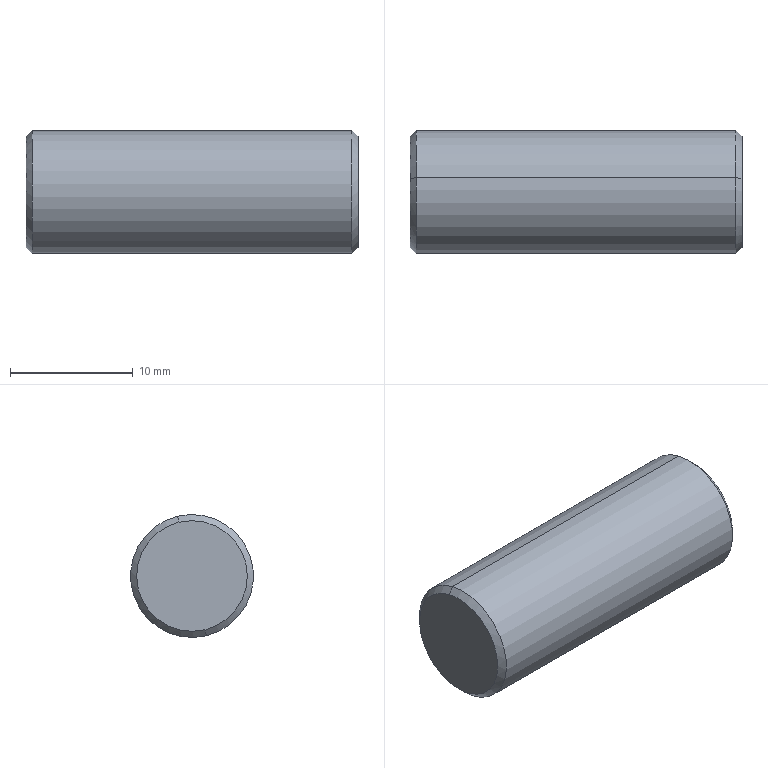Component | SolidWorks | STB-08-015-1 | 1 solid | 8 faces | box 27 x 10 x 10 mm | volume 2113 mm3 | cone 4 | cylinder 2 | plane 2 | commonest cylinder face diameters 10 x2
build123d program:
from build123d import *

# Parameters (mm, degrees)
SKETCH1_R           = 5
BOSS_EXTRUDE1_DEPTH = 13.5
CHAMFER1_SIZE       = 0.5


with BuildPart() as part:
    # Sketch1 → Boss-Extrude1 (new, symmetric)
    with BuildSketch(Plane(origin=(0, 0, 0), x_dir=(0, 0, -1), z_dir=(1, 0, 0))):
        Circle(SKETCH1_R)
    extrude(amount=BOSS_EXTRUDE1_DEPTH, both=True)

    # Chamfer1
    chamfer1_edges = [part.edges().sort_by_distance(p)[0] for p in [
        (-13.5, 0, 5),
        (13.5, 0, 5),
    ]]
    chamfer(chamfer1_edges, length=CHAMFER1_SIZE)


solid = part.part

# Placed as in the assembly
solid = solid.moved(Location((-241.404, 211.999, 2), (0, 0, 0)))
STEP:
#1=CARTESIAN_POINT('',(-8.973,8.388,0.251));
#2=VERTEX_POINT('',#1);
#3=CARTESIAN_POINT('',(-8.973,8.305,-0.09347));
#4=VERTEX_POINT('',#3);
#5=CARTESIAN_POINT('',(-8.973,8.346,0.07874));
#6=DIRECTION('',(1.,0.,0.));
#7=DIRECTION('',(0.,0.2348,0.972));
#8=AXIS2_PLACEMENT_3D('',#5,#6,#7);
#9=CIRCLE('',#8,0.1772);
#10=EDGE_CURVE('',#2,#4,#9,.T.);
#11=ORIENTED_EDGE('',*,*,#10,.F.);
#12=CARTESIAN_POINT('',(-8.992,8.393,0.2701));
#13=VERTEX_POINT('',#12);
#14=CARTESIAN_POINT('',(-8.973,8.388,0.251));
#15=DIRECTION('',(-0.7071,0.166,0.6873));
#16=VECTOR('',#15,39.37);
#17=LINE('',#14,#16);
#18=EDGE_CURVE('',#2,#13,#17,.T.);
#19=ORIENTED_EDGE('',*,*,#18,.T.);
#20=CARTESIAN_POINT('',(-8.992,8.3,-0.1126));
#21=VERTEX_POINT('',#20);
#22=CARTESIAN_POINT('',(-8.992,8.346,0.07874));
#23=DIRECTION('',(-1.,0.,0.));
#24=DIRECTION('',(0.,0.2348,0.972));
#25=AXIS2_PLACEMENT_3D('',#22,#23,#24);
#26=CIRCLE('',#25,0.1969);
#27=EDGE_CURVE('',#21,#13,#26,.T.);
#28=ORIENTED_EDGE('',*,*,#27,.F.);
#29=CARTESIAN_POINT('',(-8.973,8.305,-0.09347));
#30=DIRECTION('',(-0.7071,-0.166,-0.6873));
#31=VECTOR('',#30,39.37);
#32=LINE('',#29,#31);
#33=EDGE_CURVE('',#4,#21,#32,.T.);
#34=ORIENTED_EDGE('',*,*,#33,.F.);
#35=EDGE_LOOP('',(#11,#19,#28,#34));
#36=FACE_OUTER_BOUND('',#35,.T.);
#37=CARTESIAN_POINT('',(-8.973,8.346,0.07874));
#38=DIRECTION('',(-1.,0.,0.));
#39=DIRECTION('',(0.,-0.2348,-0.972));
#40=AXIS2_PLACEMENT_3D('',#37,#38,#39);
#41=CONICAL_SURFACE('',#40,0.1772,0.7854);
#42=ADVANCED_FACE('',(#36),#41,.T.);
#43=CARTESIAN_POINT('',(-10.036,8.305,-0.09347));
#44=VERTEX_POINT('',#43);
#45=CARTESIAN_POINT('',(-10.036,8.388,0.251));
#46=VERTEX_POINT('',#45);
#47=CARTESIAN_POINT('',(-10.036,8.346,0.07874));
#48=DIRECTION('',(-1.,0.,0.));
#49=DIRECTION('',(0.,0.2348,0.972));
#50=AXIS2_PLACEMENT_3D('',#47,#48,#49);
#51=CIRCLE('',#50,0.1772);
#52=EDGE_CURVE('',#44,#46,#51,.T.);
#53=ORIENTED_EDGE('',*,*,#52,.F.);
#54=CARTESIAN_POINT('',(-10.016,8.3,-0.1126));
#55=VERTEX_POINT('',#54);
#56=CARTESIAN_POINT('',(-10.016,8.3,-0.1126));
#57=DIRECTION('',(0.7071,-0.166,-0.6873));
#58=VECTOR('',#57,39.37);
#59=LINE('',#56,#58);
#60=EDGE_CURVE('',#44,#55,#59,.T.);
#61=ORIENTED_EDGE('',*,*,#60,.T.);
#62=CARTESIAN_POINT('',(-10.016,8.393,0.2701));
#63=VERTEX_POINT('',#62);
#64=CARTESIAN_POINT('',(-10.016,8.346,0.07874));
#65=DIRECTION('',(1.,0.,0.));
#66=DIRECTION('',(0.,0.2348,0.972));
#67=AXIS2_PLACEMENT_3D('',#64,#65,#66);
#68=CIRCLE('',#67,0.1969);
#69=EDGE_CURVE('',#63,#55,#68,.T.);
#70=ORIENTED_EDGE('',*,*,#69,.F.);
#71=CARTESIAN_POINT('',(-10.016,8.393,0.2701));
#72=DIRECTION('',(0.7071,0.166,0.6873));
#73=VECTOR('',#72,39.37);
#74=LINE('',#71,#73);
#75=EDGE_CURVE('',#46,#63,#74,.T.);
#76=ORIENTED_EDGE('',*,*,#75,.F.);
#77=EDGE_LOOP('',(#53,#61,#70,#76));
#78=FACE_OUTER_BOUND('',#77,.T.);
#79=CARTESIAN_POINT('',(-10.016,8.346,0.07874));
#80=DIRECTION('',(1.,0.,0.));
#81=DIRECTION('',(0.,0.2348,0.972));
#82=AXIS2_PLACEMENT_3D('',#79,#80,#81);
#83=CONICAL_SURFACE('',#82,0.1969,0.7854);
#84=ADVANCED_FACE('',(#78),#83,.T.);
#85=ORIENTED_EDGE('',*,*,#27,.T.);
#86=CARTESIAN_POINT('',(-8.973,8.393,0.2701));
#87=DIRECTION('',(-1.,0.,0.));
#88=VECTOR('',#87,39.37);
#89=LINE('',#86,#88);
#90=EDGE_CURVE('',#13,#63,#89,.T.);
#91=ORIENTED_EDGE('',*,*,#90,.T.);
#92=ORIENTED_EDGE('',*,*,#69,.T.);
#93=CARTESIAN_POINT('',(-8.973,8.3,-0.1126));
#94=DIRECTION('',(-1.,0.,0.));
#95=VECTOR('',#94,39.37);
#96=LINE('',#93,#95);
#97=EDGE_CURVE('',#21,#55,#96,.T.);
#98=ORIENTED_EDGE('',*,*,#97,.F.);
#99=EDGE_LOOP('',(#85,#91,#92,#98));
#100=FACE_OUTER_BOUND('',#99,.T.);
#101=CARTESIAN_POINT('',(-8.973,8.346,0.07874));
#102=DIRECTION('',(-1.,0.,0.));
#103=DIRECTION('',(0.,-0.2348,-0.972));
#104=AXIS2_PLACEMENT_3D('',#101,#102,#103);
#105=CYLINDRICAL_SURFACE('',#104,0.1969);
#106=ADVANCED_FACE('',(#100),#105,.T.);
#107=ORIENTED_EDGE('',*,*,#90,.F.);
#108=CARTESIAN_POINT('',(-8.992,8.346,0.07874));
#109=DIRECTION('',(-1.,0.,0.));
#110=DIRECTION('',(0.,0.2348,0.972));
#111=AXIS2_PLACEMENT_3D('',#108,#109,#110);
#112=CIRCLE('',#111,0.1969);
#113=EDGE_CURVE('',#13,#21,#112,.T.);
#114=ORIENTED_EDGE('',*,*,#113,.T.);
#115=ORIENTED_EDGE('',*,*,#97,.T.);
#116=CARTESIAN_POINT('',(-10.016,8.346,0.07874));
#117=DIRECTION('',(1.,0.,0.));
#118=DIRECTION('',(0.,0.2348,0.972));
#119=AXIS2_PLACEMENT_3D('',#116,#117,#118);
#120=CIRCLE('',#119,0.1969);
#121=EDGE_CURVE('',#55,#63,#120,.T.);
#122=ORIENTED_EDGE('',*,*,#121,.T.);
#123=EDGE_LOOP('',(#107,#114,#115,#122));
#124=FACE_OUTER_BOUND('',#123,.T.);
#125=CARTESIAN_POINT('',(-8.973,8.346,0.07874));
#126=DIRECTION('',(-1.,0.,0.));
#127=DIRECTION('',(0.,-0.2348,-0.972));
#128=AXIS2_PLACEMENT_3D('',#125,#126,#127);
#129=CYLINDRICAL_SURFACE('',#128,0.1969);
#130=ADVANCED_FACE('',(#124),#129,.T.);
#131=CARTESIAN_POINT('',(-8.973,8.346,0.07874));
#132=DIRECTION('',(1.,0.,0.));
#133=DIRECTION('',(0.,0.2348,0.972));
#134=AXIS2_PLACEMENT_3D('',#131,#132,#133);
#135=CIRCLE('',#134,0.1772);
#136=EDGE_CURVE('',#4,#2,#135,.T.);
#137=ORIENTED_EDGE('',*,*,#136,.T.);
#138=ORIENTED_EDGE('',*,*,#10,.T.);
#139=EDGE_LOOP('',(#137,#138));
#140=FACE_OUTER_BOUND('',#139,.T.);
#141=CARTESIAN_POINT('',(-8.973,8.346,0.07874));
#142=DIRECTION('',(1.,0.,0.));
#143=DIRECTION('',(0.,0.2348,0.972));
#144=AXIS2_PLACEMENT_3D('',#141,#142,#143);
#145=PLANE('',#144);
#146=ADVANCED_FACE('',(#140),#145,.T.);
#147=CARTESIAN_POINT('',(-10.036,8.346,0.07874));
#148=DIRECTION('',(-1.,0.,0.));
#149=DIRECTION('',(0.,0.2348,0.972));
#150=AXIS2_PLACEMENT_3D('',#147,#148,#149);
#151=CIRCLE('',#150,0.1772);
#152=EDGE_CURVE('',#46,#44,#151,.T.);
#153=ORIENTED_EDGE('',*,*,#152,.T.);
#154=ORIENTED_EDGE('',*,*,#52,.T.);
#155=EDGE_LOOP('',(#153,#154));
#156=FACE_OUTER_BOUND('',#155,.T.);
#157=CARTESIAN_POINT('',(-10.036,8.346,0.07874));
#158=DIRECTION('',(1.,0.,0.));
#159=DIRECTION('',(0.,0.2348,0.972));
#160=AXIS2_PLACEMENT_3D('',#157,#158,#159);
#161=PLANE('',#160);
#162=ADVANCED_FACE('',(#156),#161,.F.);
#163=ORIENTED_EDGE('',*,*,#60,.F.);
#164=ORIENTED_EDGE('',*,*,#152,.F.);
#165=ORIENTED_EDGE('',*,*,#75,.T.);
#166=ORIENTED_EDGE('',*,*,#121,.F.);
#167=EDGE_LOOP('',(#163,#164,#165,#166));
#168=FACE_OUTER_BOUND('',#167,.T.);
#169=CARTESIAN_POINT('',(-10.016,8.346,0.07874));
#170=DIRECTION('',(1.,0.,0.));
#171=DIRECTION('',(0.,0.2348,0.972));
#172=AXIS2_PLACEMENT_3D('',#169,#170,#171);
#173=CONICAL_SURFACE('',#172,0.1969,0.7854);
#174=ADVANCED_FACE('',(#168),#173,.T.);
#175=ORIENTED_EDGE('',*,*,#18,.F.);
#176=ORIENTED_EDGE('',*,*,#136,.F.);
#177=ORIENTED_EDGE('',*,*,#33,.T.);
#178=ORIENTED_EDGE('',*,*,#113,.F.);
#179=EDGE_LOOP('',(#175,#176,#177,#178));
#180=FACE_OUTER_BOUND('',#179,.T.);
#181=CARTESIAN_POINT('',(-8.973,8.346,0.07874));
#182=DIRECTION('',(-1.,0.,0.));
#183=DIRECTION('',(0.,-0.2348,-0.972));
#184=AXIS2_PLACEMENT_3D('',#181,#182,#183);
#185=CONICAL_SURFACE('',#184,0.1772,0.7854);
#186=ADVANCED_FACE('',(#180),#185,.T.);
#187=CLOSED_SHELL('',(#42,#84,#106,#130,#146,#162,#174,#186));
#188=MANIFOLD_SOLID_BREP('',#187);
#189=CARTESIAN_POINT('',(0.,0.,0.));
#190=DIRECTION('',(0.,0.,1.));
#191=DIRECTION('',(1.,0.,0.));
#192=AXIS2_PLACEMENT_3D('',#189,#190,#191);
#193=(LENGTH_UNIT()NAMED_UNIT(*)SI_UNIT($,.METRE.));
#194=LENGTH_MEASURE_WITH_UNIT(LENGTH_MEASURE(0.0254),#193);
#195=DIMENSIONAL_EXPONENTS(1.,0.,0.,0.,0.,0.,0.);
#196=(CONVERSION_BASED_UNIT('',#194)LENGTH_UNIT()NAMED_UNIT(#195));
#197=UNCERTAINTY_MEASURE_WITH_UNIT(LENGTH_MEASURE(0.00001),#196,'','');
#198=(NAMED_UNIT(*)PLANE_ANGLE_UNIT()SI_UNIT($,.RADIAN.));
#199=(NAMED_UNIT(*)SI_UNIT($,.STERADIAN.)SOLID_ANGLE_UNIT());
#200=(GEOMETRIC_REPRESENTATION_CONTEXT(3)GLOBAL_UNCERTAINTY_ASSIGNED_CONTEXT((#197))GLOBAL_UNIT_ASSIGNED_CONTEXT((#196,#198,#199))REPRESENTATION_CONTEXT('',''));
#201=ADVANCED_BREP_SHAPE_REPRESENTATION('',(#188,#192),#200);
#202=COLOUR_RGB('',0.7922,0.8196,0.9333);
#203=FILL_AREA_STYLE_COLOUR('',#202);
#204=FILL_AREA_STYLE('',(#203));
#205=SURFACE_STYLE_FILL_AREA(#204);
#206=SURFACE_SIDE_STYLE('',(#205));
#207=SURFACE_STYLE_USAGE(.BOTH.,#206);
#208=PRESENTATION_STYLE_ASSIGNMENT((#207));
#209=STYLED_ITEM('',(#208),#188);
#210=(LENGTH_UNIT()NAMED_UNIT(*)SI_UNIT($,.METRE.));
#211=LENGTH_MEASURE_WITH_UNIT(LENGTH_MEASURE(0.0254),#210);
#212=DIMENSIONAL_EXPONENTS(1.,0.,0.,0.,0.,0.,0.);
#213=(CONVERSION_BASED_UNIT('',#211)LENGTH_UNIT()NAMED_UNIT(#212));
#214=UNCERTAINTY_MEASURE_WITH_UNIT(LENGTH_MEASURE(0.00001),#213,'','');
#215=(NAMED_UNIT(*)PLANE_ANGLE_UNIT()SI_UNIT($,.RADIAN.));
#216=(NAMED_UNIT(*)SI_UNIT($,.STERADIAN.)SOLID_ANGLE_UNIT());
#217=(GEOMETRIC_REPRESENTATION_CONTEXT(3)GLOBAL_UNCERTAINTY_ASSIGNED_CONTEXT((#214))GLOBAL_UNIT_ASSIGNED_CONTEXT((#213,#215,#216))REPRESENTATION_CONTEXT('',''));
#218=MECHANICAL_DESIGN_GEOMETRIC_PRESENTATION_REPRESENTATION('',(#209),#217);
#219=PRESENTATION_LAYER_ASSIGNMENT('','',(#209));